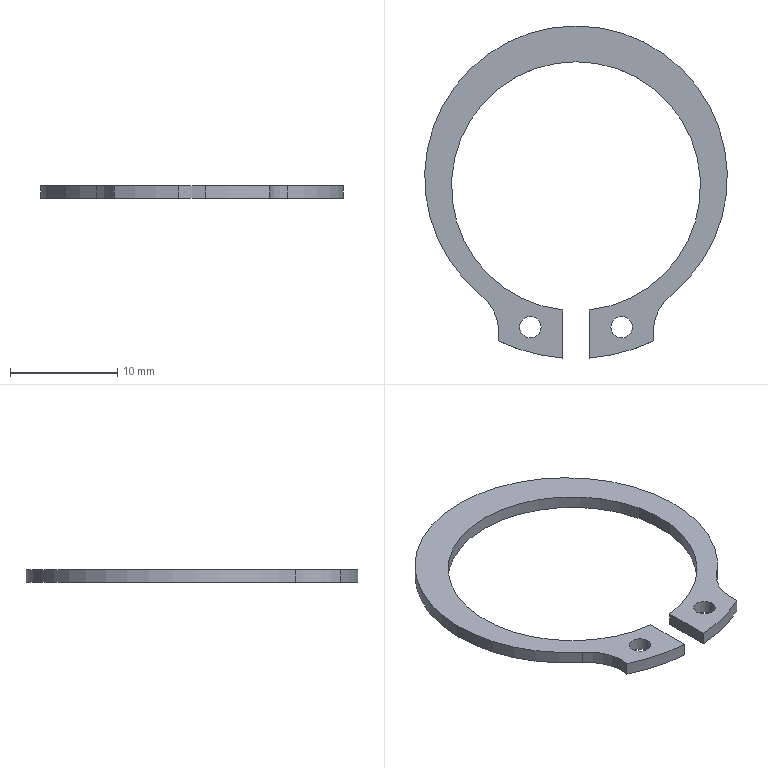Component | NX | RETAINING_RING | 1 solid | 12 faces | box 28.2 x 30.93 x 1.2 mm | volume 273 mm3 | cylinder 8 | plane 4 | commonest cylinder face diameters 2 x2 9 x2 33.76 x2 28.2 x1 23.2 x1
STEP:
#1=CARTESIAN_POINT('',(0.,0.,0.));
#2=DIRECTION('',(0.,0.,1.));
#3=DIRECTION('',(1.,0.,0.));
#4=AXIS2_PLACEMENT_3D('',#1,#2,#3);
#5=CARTESIAN_POINT('',(-594.925,295.052,-700.));
#6=VERTEX_POINT('',#5);
#7=CARTESIAN_POINT('',(-593.925,295.052,-700.));
#8=DIRECTION('',(0.,0.,1.));
#9=DIRECTION('',(-1.,0.,0.));
#10=AXIS2_PLACEMENT_3D('',#7,#8,#9);
#11=CIRCLE('',#10,1.);
#12=CARTESIAN_POINT('',(-593.925,295.052,-700.));
#13=DIRECTION('',(0.,0.,-1.));
#14=DIRECTION('',(1.,0.,0.));
#15=AXIS2_PLACEMENT_3D('',#12,#13,#14);
#16=CYLINDRICAL_SURFACE('',#15,1.);
#17=CARTESIAN_POINT('',(9.425,0.));
#18=DIRECTION('',(-1.,0.));
#19=VECTOR('',#18,1.);
#20=LINE('',#17,#19);
#21=(GEOMETRIC_REPRESENTATION_CONTEXT(2)PARAMETRIC_REPRESENTATION_CONTEXT()REPRESENTATION_CONTEXT('',''));
#22=DEFINITIONAL_REPRESENTATION('',(#20),#21);
#23=PCURVE('',#16,#22);
#24=CARTESIAN_POINT('',(-598.175,308.181,-700.));
#25=DIRECTION('',(0.,0.,1.));
#26=DIRECTION('',(-1.,0.,0.));
#27=AXIS2_PLACEMENT_3D('',#24,#25,#26);
#28=PLANE('',#27);
#29=CARTESIAN_POINT('',(-4.25,13.129));
#30=DIRECTION('',(1.,0.));
#31=AXIS2_PLACEMENT_2D('',#29,#30);
#32=CIRCLE('',#31,1.);
#33=(GEOMETRIC_REPRESENTATION_CONTEXT(2)PARAMETRIC_REPRESENTATION_CONTEXT()REPRESENTATION_CONTEXT('',''));
#34=DEFINITIONAL_REPRESENTATION('',(#32),#33);
#35=PCURVE('',#28,#34);
#36=SURFACE_CURVE('',#11,(#23,#35),.PCURVE_S1.);
#37=EDGE_CURVE('',#6,#6,#36,.T.);
#38=ORIENTED_EDGE('',*,*,#37,.F.);
#39=CARTESIAN_POINT('',(-594.925,295.052,-701.2));
#40=VERTEX_POINT('',#39);
#41=CARTESIAN_POINT('',(-594.925,295.052,-700.));
#42=CARTESIAN_POINT('',(-594.925,295.052,-701.2));
#43=B_SPLINE_CURVE_WITH_KNOTS('',1,(#41,#42),.UNSPECIFIED.,.F.,.F.,(2,2),(0.,1.2),.PIECEWISE_BEZIER_KNOTS.);
#44=CARTESIAN_POINT('',(9.425,0.));
#45=DIRECTION('',(0.,1.));
#46=VECTOR('',#45,1.);
#47=LINE('',#44,#46);
#48=(GEOMETRIC_REPRESENTATION_CONTEXT(2)PARAMETRIC_REPRESENTATION_CONTEXT()REPRESENTATION_CONTEXT('',''));
#49=DEFINITIONAL_REPRESENTATION('',(#47),#48);
#50=PCURVE('',#16,#49);
#51=CARTESIAN_POINT('',(3.142,0.));
#52=DIRECTION('',(0.,1.));
#53=VECTOR('',#52,1.);
#54=LINE('',#51,#53);
#55=(GEOMETRIC_REPRESENTATION_CONTEXT(2)PARAMETRIC_REPRESENTATION_CONTEXT()REPRESENTATION_CONTEXT('',''));
#56=DEFINITIONAL_REPRESENTATION('',(#54),#55);
#57=PCURVE('',#16,#56);
#58=SEAM_CURVE('',#43,(#50,#57),.PCURVE_S1.);
#59=EDGE_CURVE('',#6,#40,#58,.T.);
#60=ORIENTED_EDGE('',*,*,#59,.T.);
#61=CARTESIAN_POINT('',(-593.925,295.052,-701.2));
#62=DIRECTION('',(0.,0.,1.));
#63=DIRECTION('',(-1.,0.,0.));
#64=AXIS2_PLACEMENT_3D('',#61,#62,#63);
#65=CIRCLE('',#64,1.);
#66=CARTESIAN_POINT('',(9.425,1.2));
#67=DIRECTION('',(-1.,0.));
#68=VECTOR('',#67,1.);
#69=LINE('',#66,#68);
#70=(GEOMETRIC_REPRESENTATION_CONTEXT(2)PARAMETRIC_REPRESENTATION_CONTEXT()REPRESENTATION_CONTEXT('',''));
#71=DEFINITIONAL_REPRESENTATION('',(#69),#70);
#72=PCURVE('',#16,#71);
#73=CARTESIAN_POINT('',(-598.175,308.181,-701.2));
#74=DIRECTION('',(0.,0.,1.));
#75=DIRECTION('',(-1.,0.,0.));
#76=AXIS2_PLACEMENT_3D('',#73,#74,#75);
#77=PLANE('',#76);
#78=CARTESIAN_POINT('',(-4.25,13.129));
#79=DIRECTION('',(1.,0.));
#80=AXIS2_PLACEMENT_2D('',#78,#79);
#81=CIRCLE('',#80,1.);
#82=(GEOMETRIC_REPRESENTATION_CONTEXT(2)PARAMETRIC_REPRESENTATION_CONTEXT()REPRESENTATION_CONTEXT('',''));
#83=DEFINITIONAL_REPRESENTATION('',(#81),#82);
#84=PCURVE('',#77,#83);
#85=SURFACE_CURVE('',#65,(#72,#84),.PCURVE_S1.);
#86=EDGE_CURVE('',#40,#40,#85,.T.);
#87=ORIENTED_EDGE('',*,*,#86,.T.);
#88=ORIENTED_EDGE('',*,*,#59,.F.);
#89=EDGE_LOOP('',(#38,#60,#87,#88));
#90=FACE_BOUND('',#89,.F.);
#91=ADVANCED_FACE('',(#90),#16,.F.);
#92=CARTESIAN_POINT('',(-601.425,295.052,-700.));
#93=VERTEX_POINT('',#92);
#94=CARTESIAN_POINT('',(-602.425,295.052,-700.));
#95=DIRECTION('',(0.,0.,1.));
#96=DIRECTION('',(1.,0.,0.));
#97=AXIS2_PLACEMENT_3D('',#94,#95,#96);
#98=CIRCLE('',#97,1.);
#99=CARTESIAN_POINT('',(-602.425,295.052,-700.));
#100=DIRECTION('',(0.,0.,-1.));
#101=DIRECTION('',(1.,0.,0.));
#102=AXIS2_PLACEMENT_3D('',#99,#100,#101);
#103=CYLINDRICAL_SURFACE('',#102,1.);
#104=CARTESIAN_POINT('',(6.283,0.));
#105=DIRECTION('',(-1.,0.));
#106=VECTOR('',#105,1.);
#107=LINE('',#104,#106);
#108=(GEOMETRIC_REPRESENTATION_CONTEXT(2)PARAMETRIC_REPRESENTATION_CONTEXT()REPRESENTATION_CONTEXT('',''));
#109=DEFINITIONAL_REPRESENTATION('',(#107),#108);
#110=PCURVE('',#103,#109);
#111=CARTESIAN_POINT('',(4.25,13.129));
#112=DIRECTION('',(-1.,0.));
#113=AXIS2_PLACEMENT_2D('',#111,#112);
#114=CIRCLE('',#113,1.);
#115=(GEOMETRIC_REPRESENTATION_CONTEXT(2)PARAMETRIC_REPRESENTATION_CONTEXT()REPRESENTATION_CONTEXT('',''));
#116=DEFINITIONAL_REPRESENTATION('',(#114),#115);
#117=PCURVE('',#28,#116);
#118=SURFACE_CURVE('',#98,(#110,#117),.PCURVE_S1.);
#119=EDGE_CURVE('',#93,#93,#118,.T.);
#120=ORIENTED_EDGE('',*,*,#119,.F.);
#121=CARTESIAN_POINT('',(-601.425,295.052,-701.2));
#122=VERTEX_POINT('',#121);
#123=CARTESIAN_POINT('',(-601.425,295.052,-700.));
#124=CARTESIAN_POINT('',(-601.425,295.052,-701.2));
#125=B_SPLINE_CURVE_WITH_KNOTS('',1,(#123,#124),.UNSPECIFIED.,.F.,.F.,(2,2),(0.,1.2),.PIECEWISE_BEZIER_KNOTS.);
#126=CARTESIAN_POINT('',(6.283,0.));
#127=DIRECTION('',(0.,1.));
#128=VECTOR('',#127,1.);
#129=LINE('',#126,#128);
#130=(GEOMETRIC_REPRESENTATION_CONTEXT(2)PARAMETRIC_REPRESENTATION_CONTEXT()REPRESENTATION_CONTEXT('',''));
#131=DEFINITIONAL_REPRESENTATION('',(#129),#130);
#132=PCURVE('',#103,#131);
#133=CARTESIAN_POINT('',(0.,0.));
#134=DIRECTION('',(0.,1.));
#135=VECTOR('',#134,1.);
#136=LINE('',#133,#135);
#137=(GEOMETRIC_REPRESENTATION_CONTEXT(2)PARAMETRIC_REPRESENTATION_CONTEXT()REPRESENTATION_CONTEXT('',''));
#138=DEFINITIONAL_REPRESENTATION('',(#136),#137);
#139=PCURVE('',#103,#138);
#140=SEAM_CURVE('',#125,(#132,#139),.PCURVE_S1.);
#141=EDGE_CURVE('',#93,#122,#140,.T.);
#142=ORIENTED_EDGE('',*,*,#141,.T.);
#143=CARTESIAN_POINT('',(-602.425,295.052,-701.2));
#144=DIRECTION('',(0.,0.,1.));
#145=DIRECTION('',(1.,0.,0.));
#146=AXIS2_PLACEMENT_3D('',#143,#144,#145);
#147=CIRCLE('',#146,1.);
#148=CARTESIAN_POINT('',(6.283,1.2));
#149=DIRECTION('',(-1.,0.));
#150=VECTOR('',#149,1.);
#151=LINE('',#148,#150);
#152=(GEOMETRIC_REPRESENTATION_CONTEXT(2)PARAMETRIC_REPRESENTATION_CONTEXT()REPRESENTATION_CONTEXT('',''));
#153=DEFINITIONAL_REPRESENTATION('',(#151),#152);
#154=PCURVE('',#103,#153);
#155=CARTESIAN_POINT('',(4.25,13.129));
#156=DIRECTION('',(-1.,0.));
#157=AXIS2_PLACEMENT_2D('',#155,#156);
#158=CIRCLE('',#157,1.);
#159=(GEOMETRIC_REPRESENTATION_CONTEXT(2)PARAMETRIC_REPRESENTATION_CONTEXT()REPRESENTATION_CONTEXT('',''));
#160=DEFINITIONAL_REPRESENTATION('',(#158),#159);
#161=PCURVE('',#77,#160);
#162=SURFACE_CURVE('',#147,(#154,#161),.PCURVE_S1.);
#163=EDGE_CURVE('',#122,#122,#162,.T.);
#164=ORIENTED_EDGE('',*,*,#163,.T.);
#165=ORIENTED_EDGE('',*,*,#141,.F.);
#166=EDGE_LOOP('',(#120,#142,#164,#165));
#167=FACE_BOUND('',#166,.F.);
#168=ADVANCED_FACE('',(#167),#103,.F.);
#169=CARTESIAN_POINT('',(-589.318,298.04,-700.));
#170=VERTEX_POINT('',#169);
#171=CARTESIAN_POINT('',(-607.032,298.04,-700.));
#172=VERTEX_POINT('',#171);
#173=CARTESIAN_POINT('',(-598.175,309.011,-700.));
#174=DIRECTION('',(0.,0.,1.));
#175=DIRECTION('',(1.,0.,0.));
#176=AXIS2_PLACEMENT_3D('',#173,#174,#175);
#177=CIRCLE('',#176,14.1);
#178=CARTESIAN_POINT('',(-598.175,309.011,-700.));
#179=DIRECTION('',(0.,0.,-1.));
#180=DIRECTION('',(1.,0.,0.));
#181=AXIS2_PLACEMENT_3D('',#178,#179,#180);
#182=CYLINDRICAL_SURFACE('',#181,14.1);
#183=CARTESIAN_POINT('',(12.566,0.));
#184=DIRECTION('',(-1.,0.));
#185=VECTOR('',#184,1.);
#186=LINE('',#183,#185);
#187=(GEOMETRIC_REPRESENTATION_CONTEXT(2)PARAMETRIC_REPRESENTATION_CONTEXT()REPRESENTATION_CONTEXT('',''));
#188=DEFINITIONAL_REPRESENTATION('',(#186),#187);
#189=PCURVE('',#182,#188);
#190=CARTESIAN_POINT('',(0.,-0.83));
#191=DIRECTION('',(-1.,0.));
#192=AXIS2_PLACEMENT_2D('',#190,#191);
#193=CIRCLE('',#192,14.1);
#194=(GEOMETRIC_REPRESENTATION_CONTEXT(2)PARAMETRIC_REPRESENTATION_CONTEXT()REPRESENTATION_CONTEXT('',''));
#195=DEFINITIONAL_REPRESENTATION('',(#193),#194);
#196=PCURVE('',#28,#195);
#197=SURFACE_CURVE('',#177,(#189,#196),.PCURVE_S1.);
#198=EDGE_CURVE('',#170,#172,#197,.T.);
#199=ORIENTED_EDGE('',*,*,#198,.F.);
#200=CARTESIAN_POINT('',(-589.318,298.04,-701.2));
#201=VERTEX_POINT('',#200);
#202=CARTESIAN_POINT('',(-589.318,298.04,-700.));
#203=DIRECTION('',(0.,0.,-1.));
#204=VECTOR('',#203,1.);
#205=LINE('',#202,#204);
#206=CARTESIAN_POINT('',(7.175,0.));
#207=DIRECTION('',(0.,1.));
#208=VECTOR('',#207,1.);
#209=LINE('',#206,#208);
#210=(GEOMETRIC_REPRESENTATION_CONTEXT(2)PARAMETRIC_REPRESENTATION_CONTEXT()REPRESENTATION_CONTEXT('',''));
#211=DEFINITIONAL_REPRESENTATION('',(#209),#210);
#212=PCURVE('',#182,#211);
#213=CARTESIAN_POINT('',(-586.492,294.539,-700.));
#214=DIRECTION('',(0.,0.,-1.));
#215=DIRECTION('',(1.,0.,0.));
#216=AXIS2_PLACEMENT_3D('',#213,#214,#215);
#217=CYLINDRICAL_SURFACE('',#216,4.5);
#218=CARTESIAN_POINT('',(4.033,0.));
#219=DIRECTION('',(0.,1.));
#220=VECTOR('',#219,1.);
#221=LINE('',#218,#220);
#222=(GEOMETRIC_REPRESENTATION_CONTEXT(2)PARAMETRIC_REPRESENTATION_CONTEXT()REPRESENTATION_CONTEXT('',''));
#223=DEFINITIONAL_REPRESENTATION('',(#221),#222);
#224=PCURVE('',#217,#223);
#225=SURFACE_CURVE('',#205,(#212,#224),.PCURVE_S1.);
#226=EDGE_CURVE('',#170,#201,#225,.T.);
#227=ORIENTED_EDGE('',*,*,#226,.T.);
#228=CARTESIAN_POINT('',(-607.032,298.04,-701.2));
#229=VERTEX_POINT('',#228);
#230=CARTESIAN_POINT('',(-598.175,309.011,-701.2));
#231=DIRECTION('',(0.,0.,1.));
#232=DIRECTION('',(1.,0.,0.));
#233=AXIS2_PLACEMENT_3D('',#230,#231,#232);
#234=CIRCLE('',#233,14.1);
#235=CARTESIAN_POINT('',(12.566,1.2));
#236=DIRECTION('',(-1.,0.));
#237=VECTOR('',#236,1.);
#238=LINE('',#235,#237);
#239=(GEOMETRIC_REPRESENTATION_CONTEXT(2)PARAMETRIC_REPRESENTATION_CONTEXT()REPRESENTATION_CONTEXT('',''));
#240=DEFINITIONAL_REPRESENTATION('',(#238),#239);
#241=PCURVE('',#182,#240);
#242=CARTESIAN_POINT('',(0.,-0.83));
#243=DIRECTION('',(-1.,0.));
#244=AXIS2_PLACEMENT_2D('',#242,#243);
#245=CIRCLE('',#244,14.1);
#246=(GEOMETRIC_REPRESENTATION_CONTEXT(2)PARAMETRIC_REPRESENTATION_CONTEXT()REPRESENTATION_CONTEXT('',''));
#247=DEFINITIONAL_REPRESENTATION('',(#245),#246);
#248=PCURVE('',#77,#247);
#249=SURFACE_CURVE('',#234,(#241,#248),.PCURVE_S1.);
#250=EDGE_CURVE('',#201,#229,#249,.T.);
#251=ORIENTED_EDGE('',*,*,#250,.T.);
#252=CARTESIAN_POINT('',(-607.032,298.04,-700.));
#253=DIRECTION('',(0.,0.,-1.));
#254=VECTOR('',#253,1.);
#255=LINE('',#252,#254);
#256=CARTESIAN_POINT('',(2.25,0.));
#257=DIRECTION('',(0.,1.));
#258=VECTOR('',#257,1.);
#259=LINE('',#256,#258);
#260=(GEOMETRIC_REPRESENTATION_CONTEXT(2)PARAMETRIC_REPRESENTATION_CONTEXT()REPRESENTATION_CONTEXT('',''));
#261=DEFINITIONAL_REPRESENTATION('',(#259),#260);
#262=PCURVE('',#182,#261);
#263=CARTESIAN_POINT('',(-609.859,294.539,-700.));
#264=DIRECTION('',(0.,0.,-1.));
#265=DIRECTION('',(1.,0.,0.));
#266=AXIS2_PLACEMENT_3D('',#263,#264,#265);
#267=CYLINDRICAL_SURFACE('',#266,4.5);
#268=CARTESIAN_POINT('',(5.392,0.));
#269=DIRECTION('',(0.,1.));
#270=VECTOR('',#269,1.);
#271=LINE('',#268,#270);
#272=(GEOMETRIC_REPRESENTATION_CONTEXT(2)PARAMETRIC_REPRESENTATION_CONTEXT()REPRESENTATION_CONTEXT('',''));
#273=DEFINITIONAL_REPRESENTATION('',(#271),#272);
#274=PCURVE('',#267,#273);
#275=SURFACE_CURVE('',#255,(#262,#274),.PCURVE_S1.);
#276=EDGE_CURVE('',#172,#229,#275,.T.);
#277=ORIENTED_EDGE('',*,*,#276,.F.);
#278=EDGE_LOOP('',(#199,#227,#251,#277));
#279=FACE_BOUND('',#278,.T.);
#280=ADVANCED_FACE('',(#279),#182,.T.);
#281=ORIENTED_EDGE('',*,*,#226,.T.);
#282=CARTESIAN_POINT('',(-590.925,293.768,-701.2));
#283=VERTEX_POINT('',#282);
#284=CARTESIAN_POINT('',(-586.492,294.539,-701.2));
#285=DIRECTION('',(0.,0.,-1.));
#286=DIRECTION('',(-1.,0.,0.));
#287=AXIS2_PLACEMENT_3D('',#284,#285,#286);
#288=CIRCLE('',#287,4.5);
#289=CARTESIAN_POINT('',(-3.142,1.2));
#290=DIRECTION('',(1.,0.));
#291=VECTOR('',#290,1.);
#292=LINE('',#289,#291);
#293=(GEOMETRIC_REPRESENTATION_CONTEXT(2)PARAMETRIC_REPRESENTATION_CONTEXT()REPRESENTATION_CONTEXT('',''));
#294=DEFINITIONAL_REPRESENTATION('',(#292),#293);
#295=PCURVE('',#217,#294);
#296=CARTESIAN_POINT('',(-7.183,13.643));
#297=CARTESIAN_POINT('',(-7.183,5.848));
#298=CARTESIAN_POINT('',(-13.933,9.746));
#299=CARTESIAN_POINT('',(-20.683,13.643));
#300=CARTESIAN_POINT('',(-13.933,17.54));
#301=CARTESIAN_POINT('',(-7.183,21.437));
#302=CARTESIAN_POINT('',(-7.183,13.643));
#303=(BOUNDED_CURVE()B_SPLINE_CURVE(2,(#296,#297,#298,#299,#300,#301,#302),.UNSPECIFIED.,.T.,.F.)B_SPLINE_CURVE_WITH_KNOTS((1,2,2,2,2,1),(-2.094,0.,2.094,4.189,6.283,8.378),.UNSPECIFIED.)CURVE()GEOMETRIC_REPRESENTATION_ITEM()RATIONAL_B_SPLINE_CURVE((1.,0.5,1.,0.5,1.,0.5,1.))REPRESENTATION_ITEM(''));
#304=(GEOMETRIC_REPRESENTATION_CONTEXT(2)PARAMETRIC_REPRESENTATION_CONTEXT()REPRESENTATION_CONTEXT('',''));
#305=DEFINITIONAL_REPRESENTATION('',(#303),#304);
#306=PCURVE('',#77,#305);
#307=SURFACE_CURVE('',#288,(#295,#306),.PCURVE_S1.);
#308=EDGE_CURVE('',#283,#201,#307,.T.);
#309=ORIENTED_EDGE('',*,*,#308,.F.);
#310=CARTESIAN_POINT('',(-590.925,293.768,-700.));
#311=VERTEX_POINT('',#310);
#312=CARTESIAN_POINT('',(-590.925,293.768,-700.));
#313=DIRECTION('',(0.,0.,-1.));
#314=VECTOR('',#313,1.);
#315=LINE('',#312,#314);
#316=CARTESIAN_POINT('',(2.969,0.));
#317=DIRECTION('',(0.,1.));
#318=VECTOR('',#317,1.);
#319=LINE('',#316,#318);
#320=(GEOMETRIC_REPRESENTATION_CONTEXT(2)PARAMETRIC_REPRESENTATION_CONTEXT()REPRESENTATION_CONTEXT('',''));
#321=DEFINITIONAL_REPRESENTATION('',(#319),#320);
#322=PCURVE('',#217,#321);
#323=CARTESIAN_POINT('',(-598.175,309.011,-700.));
#324=DIRECTION('',(0.,0.,-1.));
#325=DIRECTION('',(1.,0.,0.));
#326=AXIS2_PLACEMENT_3D('',#323,#324,#325);
#327=CYLINDRICAL_SURFACE('',#326,16.88);
#328=CARTESIAN_POINT('',(1.127,0.));
#329=DIRECTION('',(0.,1.));
#330=VECTOR('',#329,1.);
#331=LINE('',#328,#330);
#332=(GEOMETRIC_REPRESENTATION_CONTEXT(2)PARAMETRIC_REPRESENTATION_CONTEXT()REPRESENTATION_CONTEXT('',''));
#333=DEFINITIONAL_REPRESENTATION('',(#331),#332);
#334=PCURVE('',#327,#333);
#335=SURFACE_CURVE('',#315,(#322,#334),.PCURVE_S1.);
#336=EDGE_CURVE('',#311,#283,#335,.T.);
#337=ORIENTED_EDGE('',*,*,#336,.F.);
#338=CARTESIAN_POINT('',(-586.492,294.539,-700.));
#339=DIRECTION('',(0.,0.,-1.));
#340=DIRECTION('',(-1.,0.,0.));
#341=AXIS2_PLACEMENT_3D('',#338,#339,#340);
#342=CIRCLE('',#341,4.5);
#343=CARTESIAN_POINT('',(-3.142,0.));
#344=DIRECTION('',(1.,0.));
#345=VECTOR('',#344,1.);
#346=LINE('',#343,#345);
#347=(GEOMETRIC_REPRESENTATION_CONTEXT(2)PARAMETRIC_REPRESENTATION_CONTEXT()REPRESENTATION_CONTEXT('',''));
#348=DEFINITIONAL_REPRESENTATION('',(#346),#347);
#349=PCURVE('',#217,#348);
#350=CARTESIAN_POINT('',(-7.183,13.643));
#351=CARTESIAN_POINT('',(-7.183,5.848));
#352=CARTESIAN_POINT('',(-13.933,9.746));
#353=CARTESIAN_POINT('',(-20.683,13.643));
#354=CARTESIAN_POINT('',(-13.933,17.54));
#355=CARTESIAN_POINT('',(-7.183,21.437));
#356=CARTESIAN_POINT('',(-7.183,13.643));
#357=(BOUNDED_CURVE()B_SPLINE_CURVE(2,(#350,#351,#352,#353,#354,#355,#356),.UNSPECIFIED.,.T.,.F.)B_SPLINE_CURVE_WITH_KNOTS((1,2,2,2,2,1),(-2.094,0.,2.094,4.189,6.283,8.378),.UNSPECIFIED.)CURVE()GEOMETRIC_REPRESENTATION_ITEM()RATIONAL_B_SPLINE_CURVE((1.,0.5,1.,0.5,1.,0.5,1.))REPRESENTATION_ITEM(''));
#358=(GEOMETRIC_REPRESENTATION_CONTEXT(2)PARAMETRIC_REPRESENTATION_CONTEXT()REPRESENTATION_CONTEXT('',''));
#359=DEFINITIONAL_REPRESENTATION('',(#357),#358);
#360=PCURVE('',#28,#359);
#361=SURFACE_CURVE('',#342,(#349,#360),.PCURVE_S1.);
#362=EDGE_CURVE('',#311,#170,#361,.T.);
#363=ORIENTED_EDGE('',*,*,#362,.T.);
#364=EDGE_LOOP('',(#281,#309,#337,#363));
#365=FACE_BOUND('',#364,.F.);
#366=ADVANCED_FACE('',(#365),#217,.F.);
#367=CARTESIAN_POINT('',(-596.925,296.649,-700.));
#368=VERTEX_POINT('',#367);
#369=CARTESIAN_POINT('',(-596.925,296.649,-701.2));
#370=VERTEX_POINT('',#369);
#371=CARTESIAN_POINT('',(-596.925,296.649,-700.));
#372=DIRECTION('',(0.,0.,-1.));
#373=VECTOR('',#372,1.);
#374=LINE('',#371,#373);
#375=CARTESIAN_POINT('',(-598.175,308.181,-700.));
#376=DIRECTION('',(0.,0.,-1.));
#377=DIRECTION('',(1.,0.,0.));
#378=AXIS2_PLACEMENT_3D('',#375,#376,#377);
#379=CYLINDRICAL_SURFACE('',#378,11.6);
#380=CARTESIAN_POINT('',(7.746,0.));
#381=DIRECTION('',(0.,1.));
#382=VECTOR('',#381,1.);
#383=LINE('',#380,#382);
#384=(GEOMETRIC_REPRESENTATION_CONTEXT(2)PARAMETRIC_REPRESENTATION_CONTEXT()REPRESENTATION_CONTEXT('',''));
#385=DEFINITIONAL_REPRESENTATION('',(#383),#384);
#386=PCURVE('',#379,#385);
#387=CARTESIAN_POINT('',(-596.925,296.649,-700.));
#388=DIRECTION('',(1.,0.,0.));
#389=DIRECTION('',(0.,-1.,0.));
#390=AXIS2_PLACEMENT_3D('',#387,#388,#389);
#391=PLANE('',#390);
#392=CARTESIAN_POINT('',(0.,0.));
#393=DIRECTION('',(0.,1.));
#394=VECTOR('',#393,1.);
#395=LINE('',#392,#394);
#396=(GEOMETRIC_REPRESENTATION_CONTEXT(2)PARAMETRIC_REPRESENTATION_CONTEXT()REPRESENTATION_CONTEXT('',''));
#397=DEFINITIONAL_REPRESENTATION('',(#395),#396);
#398=PCURVE('',#391,#397);
#399=SURFACE_CURVE('',#374,(#386,#398),.PCURVE_S1.);
#400=EDGE_CURVE('',#368,#370,#399,.T.);
#401=ORIENTED_EDGE('',*,*,#400,.T.);
#402=CARTESIAN_POINT('',(-599.425,296.649,-701.2));
#403=VERTEX_POINT('',#402);
#404=CARTESIAN_POINT('',(-598.175,308.181,-701.2));
#405=DIRECTION('',(0.,0.,-1.));
#406=DIRECTION('',(1.,0.,0.));
#407=AXIS2_PLACEMENT_3D('',#404,#405,#406);
#408=CIRCLE('',#407,11.6);
#409=CARTESIAN_POINT('',(-0.,1.2));
#410=DIRECTION('',(1.,0.));
#411=VECTOR('',#410,1.);
#412=LINE('',#409,#411);
#413=(GEOMETRIC_REPRESENTATION_CONTEXT(2)PARAMETRIC_REPRESENTATION_CONTEXT()REPRESENTATION_CONTEXT('',''));
#414=DEFINITIONAL_REPRESENTATION('',(#412),#413);
#415=PCURVE('',#379,#414);
#416=CARTESIAN_POINT('',(-11.6,0.));
#417=CARTESIAN_POINT('',(-11.6,20.092));
#418=CARTESIAN_POINT('',(5.8,10.046));
#419=CARTESIAN_POINT('',(23.2,0.));
#420=CARTESIAN_POINT('',(5.8,-10.046));
#421=CARTESIAN_POINT('',(-11.6,-20.092));
#422=CARTESIAN_POINT('',(-11.6,0.));
#423=(BOUNDED_CURVE()B_SPLINE_CURVE(2,(#416,#417,#418,#419,#420,#421,#422),.UNSPECIFIED.,.T.,.F.)B_SPLINE_CURVE_WITH_KNOTS((1,2,2,2,2,1),(-2.094,0.,2.094,4.189,6.283,8.378),.UNSPECIFIED.)CURVE()GEOMETRIC_REPRESENTATION_ITEM()RATIONAL_B_SPLINE_CURVE((1.,0.5,1.,0.5,1.,0.5,1.))REPRESENTATION_ITEM(''));
#424=(GEOMETRIC_REPRESENTATION_CONTEXT(2)PARAMETRIC_REPRESENTATION_CONTEXT()REPRESENTATION_CONTEXT('',''));
#425=DEFINITIONAL_REPRESENTATION('',(#423),#424);
#426=PCURVE('',#77,#425);
#427=SURFACE_CURVE('',#408,(#415,#426),.PCURVE_S1.);
#428=EDGE_CURVE('',#403,#370,#427,.T.);
#429=ORIENTED_EDGE('',*,*,#428,.F.);
#430=CARTESIAN_POINT('',(-599.425,296.649,-700.));
#431=VERTEX_POINT('',#430);
#432=CARTESIAN_POINT('',(-599.425,296.649,-700.));
#433=DIRECTION('',(0.,0.,-1.));
#434=VECTOR('',#433,1.);
#435=LINE('',#432,#434);
#436=CARTESIAN_POINT('',(1.679,0.));
#437=DIRECTION('',(0.,1.));
#438=VECTOR('',#437,1.);
#439=LINE('',#436,#438);
#440=(GEOMETRIC_REPRESENTATION_CONTEXT(2)PARAMETRIC_REPRESENTATION_CONTEXT()REPRESENTATION_CONTEXT('',''));
#441=DEFINITIONAL_REPRESENTATION('',(#439),#440);
#442=PCURVE('',#379,#441);
#443=CARTESIAN_POINT('',(-599.425,296.649,-700.));
#444=DIRECTION('',(-1.,-0.,0.));
#445=DIRECTION('',(-0.,1.,0.));
#446=AXIS2_PLACEMENT_3D('',#443,#444,#445);
#447=PLANE('',#446);
#448=CARTESIAN_POINT('',(0.,0.));
#449=DIRECTION('',(0.,1.));
#450=VECTOR('',#449,1.);
#451=LINE('',#448,#450);
#452=(GEOMETRIC_REPRESENTATION_CONTEXT(2)PARAMETRIC_REPRESENTATION_CONTEXT()REPRESENTATION_CONTEXT('',''));
#453=DEFINITIONAL_REPRESENTATION('',(#451),#452);
#454=PCURVE('',#447,#453);
#455=SURFACE_CURVE('',#435,(#442,#454),.PCURVE_S1.);
#456=EDGE_CURVE('',#431,#403,#455,.T.);
#457=ORIENTED_EDGE('',*,*,#456,.F.);
#458=CARTESIAN_POINT('',(-598.175,308.181,-700.));
#459=DIRECTION('',(0.,0.,-1.));
#460=DIRECTION('',(1.,0.,0.));
#461=AXIS2_PLACEMENT_3D('',#458,#459,#460);
#462=CIRCLE('',#461,11.6);
#463=CARTESIAN_POINT('',(-0.,0.));
#464=DIRECTION('',(1.,0.));
#465=VECTOR('',#464,1.);
#466=LINE('',#463,#465);
#467=(GEOMETRIC_REPRESENTATION_CONTEXT(2)PARAMETRIC_REPRESENTATION_CONTEXT()REPRESENTATION_CONTEXT('',''));
#468=DEFINITIONAL_REPRESENTATION('',(#466),#467);
#469=PCURVE('',#379,#468);
#470=CARTESIAN_POINT('',(-11.6,0.));
#471=CARTESIAN_POINT('',(-11.6,20.092));
#472=CARTESIAN_POINT('',(5.8,10.046));
#473=CARTESIAN_POINT('',(23.2,0.));
#474=CARTESIAN_POINT('',(5.8,-10.046));
#475=CARTESIAN_POINT('',(-11.6,-20.092));
#476=CARTESIAN_POINT('',(-11.6,0.));
#477=(BOUNDED_CURVE()B_SPLINE_CURVE(2,(#470,#471,#472,#473,#474,#475,#476),.UNSPECIFIED.,.T.,.F.)B_SPLINE_CURVE_WITH_KNOTS((1,2,2,2,2,1),(-2.094,0.,2.094,4.189,6.283,8.378),.UNSPECIFIED.)CURVE()GEOMETRIC_REPRESENTATION_ITEM()RATIONAL_B_SPLINE_CURVE((1.,0.5,1.,0.5,1.,0.5,1.))REPRESENTATION_ITEM(''));
#478=(GEOMETRIC_REPRESENTATION_CONTEXT(2)PARAMETRIC_REPRESENTATION_CONTEXT()REPRESENTATION_CONTEXT('',''));
#479=DEFINITIONAL_REPRESENTATION('',(#477),#478);
#480=PCURVE('',#28,#479);
#481=SURFACE_CURVE('',#462,(#469,#480),.PCURVE_S1.);
#482=EDGE_CURVE('',#431,#368,#481,.T.);
#483=ORIENTED_EDGE('',*,*,#482,.T.);
#484=EDGE_LOOP('',(#401,#429,#457,#483));
#485=FACE_BOUND('',#484,.F.);
#486=ADVANCED_FACE('',(#485),#379,.F.);
#487=ORIENTED_EDGE('',*,*,#119,.F.);
#488=EDGE_LOOP('',(#487));
#489=FACE_BOUND('',#488,.T.);
#490=CARTESIAN_POINT('',(-599.425,292.178,-700.));
#491=VERTEX_POINT('',#490);
#492=CARTESIAN_POINT('',(-599.425,296.649,-700.));
#493=DIRECTION('',(-0.,1.,0.));
#494=VECTOR('',#493,1.);
#495=LINE('',#492,#494);
#496=CARTESIAN_POINT('',(1.25,11.532));
#497=DIRECTION('',(0.,-1.));
#498=VECTOR('',#497,1.);
#499=LINE('',#496,#498);
#500=(GEOMETRIC_REPRESENTATION_CONTEXT(2)PARAMETRIC_REPRESENTATION_CONTEXT()REPRESENTATION_CONTEXT('',''));
#501=DEFINITIONAL_REPRESENTATION('',(#499),#500);
#502=PCURVE('',#28,#501);
#503=CARTESIAN_POINT('',(0.,0.));
#504=DIRECTION('',(1.,0.));
#505=VECTOR('',#504,1.);
#506=LINE('',#503,#505);
#507=(GEOMETRIC_REPRESENTATION_CONTEXT(2)PARAMETRIC_REPRESENTATION_CONTEXT()REPRESENTATION_CONTEXT('',''));
#508=DEFINITIONAL_REPRESENTATION('',(#506),#507);
#509=PCURVE('',#447,#508);
#510=SURFACE_CURVE('',#495,(#502,#509),.PCURVE_S1.);
#511=EDGE_CURVE('',#491,#431,#510,.T.);
#512=ORIENTED_EDGE('',*,*,#511,.T.);
#513=ORIENTED_EDGE('',*,*,#482,.T.);
#514=CARTESIAN_POINT('',(-596.925,292.178,-700.));
#515=VERTEX_POINT('',#514);
#516=CARTESIAN_POINT('',(-596.925,296.649,-700.));
#517=DIRECTION('',(0.,-1.,0.));
#518=VECTOR('',#517,1.);
#519=LINE('',#516,#518);
#520=CARTESIAN_POINT('',(-1.25,11.532));
#521=DIRECTION('',(-0.,1.));
#522=VECTOR('',#521,1.);
#523=LINE('',#520,#522);
#524=(GEOMETRIC_REPRESENTATION_CONTEXT(2)PARAMETRIC_REPRESENTATION_CONTEXT()REPRESENTATION_CONTEXT('',''));
#525=DEFINITIONAL_REPRESENTATION('',(#523),#524);
#526=PCURVE('',#28,#525);
#527=CARTESIAN_POINT('',(0.,0.));
#528=DIRECTION('',(1.,0.));
#529=VECTOR('',#528,1.);
#530=LINE('',#527,#529);
#531=(GEOMETRIC_REPRESENTATION_CONTEXT(2)PARAMETRIC_REPRESENTATION_CONTEXT()REPRESENTATION_CONTEXT('',''));
#532=DEFINITIONAL_REPRESENTATION('',(#530),#531);
#533=PCURVE('',#391,#532);
#534=SURFACE_CURVE('',#519,(#526,#533),.PCURVE_S1.);
#535=EDGE_CURVE('',#368,#515,#534,.T.);
#536=ORIENTED_EDGE('',*,*,#535,.T.);
#537=CARTESIAN_POINT('',(-598.175,309.011,-700.));
#538=DIRECTION('',(0.,0.,1.));
#539=DIRECTION('',(1.,0.,0.));
#540=AXIS2_PLACEMENT_3D('',#537,#538,#539);
#541=CIRCLE('',#540,16.88);
#542=CARTESIAN_POINT('',(0.,-0.83));
#543=DIRECTION('',(-1.,0.));
#544=AXIS2_PLACEMENT_2D('',#542,#543);
#545=CIRCLE('',#544,16.88);
#546=(GEOMETRIC_REPRESENTATION_CONTEXT(2)PARAMETRIC_REPRESENTATION_CONTEXT()REPRESENTATION_CONTEXT('',''));
#547=DEFINITIONAL_REPRESENTATION('',(#545),#546);
#548=PCURVE('',#28,#547);
#549=CARTESIAN_POINT('',(6.283,0.));
#550=DIRECTION('',(-1.,0.));
#551=VECTOR('',#550,1.);
#552=LINE('',#549,#551);
#553=(GEOMETRIC_REPRESENTATION_CONTEXT(2)PARAMETRIC_REPRESENTATION_CONTEXT()REPRESENTATION_CONTEXT('',''));
#554=DEFINITIONAL_REPRESENTATION('',(#552),#553);
#555=PCURVE('',#327,#554);
#556=SURFACE_CURVE('',#541,(#548,#555),.PCURVE_S1.);
#557=EDGE_CURVE('',#515,#311,#556,.T.);
#558=ORIENTED_EDGE('',*,*,#557,.T.);
#559=ORIENTED_EDGE('',*,*,#362,.T.);
#560=ORIENTED_EDGE('',*,*,#198,.T.);
#561=CARTESIAN_POINT('',(-605.425,293.768,-700.));
#562=VERTEX_POINT('',#561);
#563=CARTESIAN_POINT('',(-609.859,294.539,-700.));
#564=DIRECTION('',(0.,0.,-1.));
#565=DIRECTION('',(1.,0.,0.));
#566=AXIS2_PLACEMENT_3D('',#563,#564,#565);
#567=CIRCLE('',#566,4.5);
#568=CARTESIAN_POINT('',(7.183,13.643));
#569=CARTESIAN_POINT('',(7.183,21.437));
#570=CARTESIAN_POINT('',(13.933,17.54));
#571=CARTESIAN_POINT('',(20.683,13.643));
#572=CARTESIAN_POINT('',(13.933,9.746));
#573=CARTESIAN_POINT('',(7.183,5.848));
#574=CARTESIAN_POINT('',(7.183,13.643));
#575=(BOUNDED_CURVE()B_SPLINE_CURVE(2,(#568,#569,#570,#571,#572,#573,#574),.UNSPECIFIED.,.T.,.F.)B_SPLINE_CURVE_WITH_KNOTS((1,2,2,2,2,1),(-2.094,0.,2.094,4.189,6.283,8.378),.UNSPECIFIED.)CURVE()GEOMETRIC_REPRESENTATION_ITEM()RATIONAL_B_SPLINE_CURVE((1.,0.5,1.,0.5,1.,0.5,1.))REPRESENTATION_ITEM(''));
#576=(GEOMETRIC_REPRESENTATION_CONTEXT(2)PARAMETRIC_REPRESENTATION_CONTEXT()REPRESENTATION_CONTEXT('',''));
#577=DEFINITIONAL_REPRESENTATION('',(#575),#576);
#578=PCURVE('',#28,#577);
#579=CARTESIAN_POINT('',(0.,0.));
#580=DIRECTION('',(1.,0.));
#581=VECTOR('',#580,1.);
#582=LINE('',#579,#581);
#583=(GEOMETRIC_REPRESENTATION_CONTEXT(2)PARAMETRIC_REPRESENTATION_CONTEXT()REPRESENTATION_CONTEXT('',''));
#584=DEFINITIONAL_REPRESENTATION('',(#582),#583);
#585=PCURVE('',#267,#584);
#586=SURFACE_CURVE('',#567,(#578,#585),.PCURVE_S1.);
#587=EDGE_CURVE('',#172,#562,#586,.T.);
#588=ORIENTED_EDGE('',*,*,#587,.T.);
#589=CARTESIAN_POINT('',(-598.175,309.011,-700.));
#590=DIRECTION('',(0.,0.,1.));
#591=DIRECTION('',(-1.,0.,0.));
#592=AXIS2_PLACEMENT_3D('',#589,#590,#591);
#593=CIRCLE('',#592,16.88);
#594=CARTESIAN_POINT('',(0.,-0.83));
#595=DIRECTION('',(1.,0.));
#596=AXIS2_PLACEMENT_2D('',#594,#595);
#597=CIRCLE('',#596,16.88);
#598=(GEOMETRIC_REPRESENTATION_CONTEXT(2)PARAMETRIC_REPRESENTATION_CONTEXT()REPRESENTATION_CONTEXT('',''));
#599=DEFINITIONAL_REPRESENTATION('',(#597),#598);
#600=PCURVE('',#28,#599);
#601=CARTESIAN_POINT('',(-598.175,309.011,-700.));
#602=DIRECTION('',(0.,0.,-1.));
#603=DIRECTION('',(1.,0.,0.));
#604=AXIS2_PLACEMENT_3D('',#601,#602,#603);
#605=CYLINDRICAL_SURFACE('',#604,16.88);
#606=CARTESIAN_POINT('',(3.142,0.));
#607=DIRECTION('',(-1.,0.));
#608=VECTOR('',#607,1.);
#609=LINE('',#606,#608);
#610=(GEOMETRIC_REPRESENTATION_CONTEXT(2)PARAMETRIC_REPRESENTATION_CONTEXT()REPRESENTATION_CONTEXT('',''));
#611=DEFINITIONAL_REPRESENTATION('',(#609),#610);
#612=PCURVE('',#605,#611);
#613=SURFACE_CURVE('',#593,(#600,#612),.PCURVE_S1.);
#614=EDGE_CURVE('',#562,#491,#613,.T.);
#615=ORIENTED_EDGE('',*,*,#614,.T.);
#616=EDGE_LOOP('',(#512,#513,#536,#558,#559,#560,#588,#615));
#617=FACE_BOUND('',#616,.T.);
#618=ORIENTED_EDGE('',*,*,#37,.F.);
#619=EDGE_LOOP('',(#618));
#620=FACE_BOUND('',#619,.T.);
#621=ADVANCED_FACE('',(#489,#617,#620),#28,.T.);
#622=ORIENTED_EDGE('',*,*,#400,.T.);
#623=CARTESIAN_POINT('',(-596.925,292.178,-701.2));
#624=VERTEX_POINT('',#623);
#625=CARTESIAN_POINT('',(-596.925,296.649,-701.2));
#626=DIRECTION('',(0.,-1.,0.));
#627=VECTOR('',#626,1.);
#628=LINE('',#625,#627);
#629=CARTESIAN_POINT('',(0.,1.2));
#630=DIRECTION('',(1.,0.));
#631=VECTOR('',#630,1.);
#632=LINE('',#629,#631);
#633=(GEOMETRIC_REPRESENTATION_CONTEXT(2)PARAMETRIC_REPRESENTATION_CONTEXT()REPRESENTATION_CONTEXT('',''));
#634=DEFINITIONAL_REPRESENTATION('',(#632),#633);
#635=PCURVE('',#391,#634);
#636=CARTESIAN_POINT('',(-1.25,11.532));
#637=DIRECTION('',(-0.,1.));
#638=VECTOR('',#637,1.);
#639=LINE('',#636,#638);
#640=(GEOMETRIC_REPRESENTATION_CONTEXT(2)PARAMETRIC_REPRESENTATION_CONTEXT()REPRESENTATION_CONTEXT('',''));
#641=DEFINITIONAL_REPRESENTATION('',(#639),#640);
#642=PCURVE('',#77,#641);
#643=SURFACE_CURVE('',#628,(#635,#642),.PCURVE_S1.);
#644=EDGE_CURVE('',#370,#624,#643,.T.);
#645=ORIENTED_EDGE('',*,*,#644,.T.);
#646=CARTESIAN_POINT('',(-596.925,292.178,-700.));
#647=DIRECTION('',(0.,0.,-1.));
#648=VECTOR('',#647,1.);
#649=LINE('',#646,#648);
#650=CARTESIAN_POINT('',(4.471,0.));
#651=DIRECTION('',(0.,1.));
#652=VECTOR('',#651,1.);
#653=LINE('',#650,#652);
#654=(GEOMETRIC_REPRESENTATION_CONTEXT(2)PARAMETRIC_REPRESENTATION_CONTEXT()REPRESENTATION_CONTEXT('',''));
#655=DEFINITIONAL_REPRESENTATION('',(#653),#654);
#656=PCURVE('',#391,#655);
#657=CARTESIAN_POINT('',(1.497,0.));
#658=DIRECTION('',(0.,1.));
#659=VECTOR('',#658,1.);
#660=LINE('',#657,#659);
#661=(GEOMETRIC_REPRESENTATION_CONTEXT(2)PARAMETRIC_REPRESENTATION_CONTEXT()REPRESENTATION_CONTEXT('',''));
#662=DEFINITIONAL_REPRESENTATION('',(#660),#661);
#663=PCURVE('',#327,#662);
#664=SURFACE_CURVE('',#649,(#656,#663),.PCURVE_S1.);
#665=EDGE_CURVE('',#515,#624,#664,.T.);
#666=ORIENTED_EDGE('',*,*,#665,.F.);
#667=ORIENTED_EDGE('',*,*,#535,.F.);
#668=EDGE_LOOP('',(#622,#645,#666,#667));
#669=FACE_BOUND('',#668,.T.);
#670=ADVANCED_FACE('',(#669),#391,.F.);
#671=ORIENTED_EDGE('',*,*,#665,.T.);
#672=CARTESIAN_POINT('',(-598.175,309.011,-701.2));
#673=DIRECTION('',(0.,0.,1.));
#674=DIRECTION('',(1.,0.,0.));
#675=AXIS2_PLACEMENT_3D('',#672,#673,#674);
#676=CIRCLE('',#675,16.88);
#677=CARTESIAN_POINT('',(6.283,1.2));
#678=DIRECTION('',(-1.,0.));
#679=VECTOR('',#678,1.);
#680=LINE('',#677,#679);
#681=(GEOMETRIC_REPRESENTATION_CONTEXT(2)PARAMETRIC_REPRESENTATION_CONTEXT()REPRESENTATION_CONTEXT('',''));
#682=DEFINITIONAL_REPRESENTATION('',(#680),#681);
#683=PCURVE('',#327,#682);
#684=CARTESIAN_POINT('',(0.,-0.83));
#685=DIRECTION('',(-1.,0.));
#686=AXIS2_PLACEMENT_2D('',#684,#685);
#687=CIRCLE('',#686,16.88);
#688=(GEOMETRIC_REPRESENTATION_CONTEXT(2)PARAMETRIC_REPRESENTATION_CONTEXT()REPRESENTATION_CONTEXT('',''));
#689=DEFINITIONAL_REPRESENTATION('',(#687),#688);
#690=PCURVE('',#77,#689);
#691=SURFACE_CURVE('',#676,(#683,#690),.PCURVE_S1.);
#692=EDGE_CURVE('',#624,#283,#691,.T.);
#693=ORIENTED_EDGE('',*,*,#692,.T.);
#694=ORIENTED_EDGE('',*,*,#336,.F.);
#695=ORIENTED_EDGE('',*,*,#557,.F.);
#696=EDGE_LOOP('',(#671,#693,#694,#695));
#697=FACE_BOUND('',#696,.T.);
#698=ADVANCED_FACE('',(#697),#327,.T.);
#699=ORIENTED_EDGE('',*,*,#587,.T.);
#700=CARTESIAN_POINT('',(-605.425,293.768,-701.2));
#701=VERTEX_POINT('',#700);
#702=CARTESIAN_POINT('',(-605.425,293.768,-700.));
#703=DIRECTION('',(0.,0.,-1.));
#704=VECTOR('',#703,1.);
#705=LINE('',#702,#704);
#706=CARTESIAN_POINT('',(6.455,0.));
#707=DIRECTION('',(0.,1.));
#708=VECTOR('',#707,1.);
#709=LINE('',#706,#708);
#710=(GEOMETRIC_REPRESENTATION_CONTEXT(2)PARAMETRIC_REPRESENTATION_CONTEXT()REPRESENTATION_CONTEXT('',''));
#711=DEFINITIONAL_REPRESENTATION('',(#709),#710);
#712=PCURVE('',#267,#711);
#713=CARTESIAN_POINT('',(2.015,0.));
#714=DIRECTION('',(0.,1.));
#715=VECTOR('',#714,1.);
#716=LINE('',#713,#715);
#717=(GEOMETRIC_REPRESENTATION_CONTEXT(2)PARAMETRIC_REPRESENTATION_CONTEXT()REPRESENTATION_CONTEXT('',''));
#718=DEFINITIONAL_REPRESENTATION('',(#716),#717);
#719=PCURVE('',#605,#718);
#720=SURFACE_CURVE('',#705,(#712,#719),.PCURVE_S1.);
#721=EDGE_CURVE('',#562,#701,#720,.T.);
#722=ORIENTED_EDGE('',*,*,#721,.T.);
#723=CARTESIAN_POINT('',(-609.859,294.539,-701.2));
#724=DIRECTION('',(0.,0.,-1.));
#725=DIRECTION('',(1.,0.,0.));
#726=AXIS2_PLACEMENT_3D('',#723,#724,#725);
#727=CIRCLE('',#726,4.5);
#728=CARTESIAN_POINT('',(0.,1.2));
#729=DIRECTION('',(1.,0.));
#730=VECTOR('',#729,1.);
#731=LINE('',#728,#730);
#732=(GEOMETRIC_REPRESENTATION_CONTEXT(2)PARAMETRIC_REPRESENTATION_CONTEXT()REPRESENTATION_CONTEXT('',''));
#733=DEFINITIONAL_REPRESENTATION('',(#731),#732);
#734=PCURVE('',#267,#733);
#735=CARTESIAN_POINT('',(7.183,13.643));
#736=CARTESIAN_POINT('',(7.183,21.437));
#737=CARTESIAN_POINT('',(13.933,17.54));
#738=CARTESIAN_POINT('',(20.683,13.643));
#739=CARTESIAN_POINT('',(13.933,9.746));
#740=CARTESIAN_POINT('',(7.183,5.848));
#741=CARTESIAN_POINT('',(7.183,13.643));
#742=(BOUNDED_CURVE()B_SPLINE_CURVE(2,(#735,#736,#737,#738,#739,#740,#741),.UNSPECIFIED.,.T.,.F.)B_SPLINE_CURVE_WITH_KNOTS((1,2,2,2,2,1),(-2.094,0.,2.094,4.189,6.283,8.378),.UNSPECIFIED.)CURVE()GEOMETRIC_REPRESENTATION_ITEM()RATIONAL_B_SPLINE_CURVE((1.,0.5,1.,0.5,1.,0.5,1.))REPRESENTATION_ITEM(''));
#743=(GEOMETRIC_REPRESENTATION_CONTEXT(2)PARAMETRIC_REPRESENTATION_CONTEXT()REPRESENTATION_CONTEXT('',''));
#744=DEFINITIONAL_REPRESENTATION('',(#742),#743);
#745=PCURVE('',#77,#744);
#746=SURFACE_CURVE('',#727,(#734,#745),.PCURVE_S1.);
#747=EDGE_CURVE('',#229,#701,#746,.T.);
#748=ORIENTED_EDGE('',*,*,#747,.F.);
#749=ORIENTED_EDGE('',*,*,#276,.F.);
#750=EDGE_LOOP('',(#699,#722,#748,#749));
#751=FACE_BOUND('',#750,.F.);
#752=ADVANCED_FACE('',(#751),#267,.F.);
#753=ORIENTED_EDGE('',*,*,#721,.T.);
#754=CARTESIAN_POINT('',(-599.425,292.178,-701.2));
#755=VERTEX_POINT('',#754);
#756=CARTESIAN_POINT('',(-598.175,309.011,-701.2));
#757=DIRECTION('',(0.,0.,1.));
#758=DIRECTION('',(-1.,0.,0.));
#759=AXIS2_PLACEMENT_3D('',#756,#757,#758);
#760=CIRCLE('',#759,16.88);
#761=CARTESIAN_POINT('',(3.142,1.2));
#762=DIRECTION('',(-1.,0.));
#763=VECTOR('',#762,1.);
#764=LINE('',#761,#763);
#765=(GEOMETRIC_REPRESENTATION_CONTEXT(2)PARAMETRIC_REPRESENTATION_CONTEXT()REPRESENTATION_CONTEXT('',''));
#766=DEFINITIONAL_REPRESENTATION('',(#764),#765);
#767=PCURVE('',#605,#766);
#768=CARTESIAN_POINT('',(0.,-0.83));
#769=DIRECTION('',(1.,0.));
#770=AXIS2_PLACEMENT_2D('',#768,#769);
#771=CIRCLE('',#770,16.88);
#772=(GEOMETRIC_REPRESENTATION_CONTEXT(2)PARAMETRIC_REPRESENTATION_CONTEXT()REPRESENTATION_CONTEXT('',''));
#773=DEFINITIONAL_REPRESENTATION('',(#771),#772);
#774=PCURVE('',#77,#773);
#775=SURFACE_CURVE('',#760,(#767,#774),.PCURVE_S1.);
#776=EDGE_CURVE('',#701,#755,#775,.T.);
#777=ORIENTED_EDGE('',*,*,#776,.T.);
#778=CARTESIAN_POINT('',(-599.425,292.178,-700.));
#779=DIRECTION('',(0.,0.,-1.));
#780=VECTOR('',#779,1.);
#781=LINE('',#778,#780);
#782=CARTESIAN_POINT('',(1.645,0.));
#783=DIRECTION('',(0.,1.));
#784=VECTOR('',#783,1.);
#785=LINE('',#782,#784);
#786=(GEOMETRIC_REPRESENTATION_CONTEXT(2)PARAMETRIC_REPRESENTATION_CONTEXT()REPRESENTATION_CONTEXT('',''));
#787=DEFINITIONAL_REPRESENTATION('',(#785),#786);
#788=PCURVE('',#605,#787);
#789=CARTESIAN_POINT('',(-4.471,0.));
#790=DIRECTION('',(0.,1.));
#791=VECTOR('',#790,1.);
#792=LINE('',#789,#791);
#793=(GEOMETRIC_REPRESENTATION_CONTEXT(2)PARAMETRIC_REPRESENTATION_CONTEXT()REPRESENTATION_CONTEXT('',''));
#794=DEFINITIONAL_REPRESENTATION('',(#792),#793);
#795=PCURVE('',#447,#794);
#796=SURFACE_CURVE('',#781,(#788,#795),.PCURVE_S1.);
#797=EDGE_CURVE('',#491,#755,#796,.T.);
#798=ORIENTED_EDGE('',*,*,#797,.F.);
#799=ORIENTED_EDGE('',*,*,#614,.F.);
#800=EDGE_LOOP('',(#753,#777,#798,#799));
#801=FACE_BOUND('',#800,.T.);
#802=ADVANCED_FACE('',(#801),#605,.T.);
#803=ORIENTED_EDGE('',*,*,#797,.T.);
#804=CARTESIAN_POINT('',(-599.425,296.649,-701.2));
#805=DIRECTION('',(-0.,1.,0.));
#806=VECTOR('',#805,1.);
#807=LINE('',#804,#806);
#808=CARTESIAN_POINT('',(0.,1.2));
#809=DIRECTION('',(1.,0.));
#810=VECTOR('',#809,1.);
#811=LINE('',#808,#810);
#812=(GEOMETRIC_REPRESENTATION_CONTEXT(2)PARAMETRIC_REPRESENTATION_CONTEXT()REPRESENTATION_CONTEXT('',''));
#813=DEFINITIONAL_REPRESENTATION('',(#811),#812);
#814=PCURVE('',#447,#813);
#815=CARTESIAN_POINT('',(1.25,11.532));
#816=DIRECTION('',(0.,-1.));
#817=VECTOR('',#816,1.);
#818=LINE('',#815,#817);
#819=(GEOMETRIC_REPRESENTATION_CONTEXT(2)PARAMETRIC_REPRESENTATION_CONTEXT()REPRESENTATION_CONTEXT('',''));
#820=DEFINITIONAL_REPRESENTATION('',(#818),#819);
#821=PCURVE('',#77,#820);
#822=SURFACE_CURVE('',#807,(#814,#821),.PCURVE_S1.);
#823=EDGE_CURVE('',#755,#403,#822,.T.);
#824=ORIENTED_EDGE('',*,*,#823,.T.);
#825=ORIENTED_EDGE('',*,*,#456,.F.);
#826=ORIENTED_EDGE('',*,*,#511,.F.);
#827=EDGE_LOOP('',(#803,#824,#825,#826));
#828=FACE_BOUND('',#827,.T.);
#829=ADVANCED_FACE('',(#828),#447,.F.);
#830=ORIENTED_EDGE('',*,*,#86,.T.);
#831=EDGE_LOOP('',(#830));
#832=FACE_BOUND('',#831,.T.);
#833=ORIENTED_EDGE('',*,*,#163,.T.);
#834=EDGE_LOOP('',(#833));
#835=FACE_BOUND('',#834,.T.);
#836=ORIENTED_EDGE('',*,*,#428,.F.);
#837=ORIENTED_EDGE('',*,*,#823,.F.);
#838=ORIENTED_EDGE('',*,*,#776,.F.);
#839=ORIENTED_EDGE('',*,*,#747,.F.);
#840=ORIENTED_EDGE('',*,*,#250,.F.);
#841=ORIENTED_EDGE('',*,*,#308,.F.);
#842=ORIENTED_EDGE('',*,*,#692,.F.);
#843=ORIENTED_EDGE('',*,*,#644,.F.);
#844=EDGE_LOOP('',(#836,#837,#838,#839,#840,#841,#842,#843));
#845=FACE_BOUND('',#844,.T.);
#846=ADVANCED_FACE('',(#832,#835,#845),#77,.F.);
#847=CLOSED_SHELL('',(#91,#168,#280,#366,#486,#621,#670,#698,#752,#802,#829,#846));
#848=MANIFOLD_SOLID_BREP('',#847);
#849=(LENGTH_UNIT()NAMED_UNIT(*)SI_UNIT(.MILLI.,.METRE.));
#850=UNCERTAINTY_MEASURE_WITH_UNIT(LENGTH_MEASURE(0.000002),#849,'','');
#851=(NAMED_UNIT(*)PLANE_ANGLE_UNIT()SI_UNIT($,.RADIAN.));
#852=(NAMED_UNIT(*)SI_UNIT($,.STERADIAN.)SOLID_ANGLE_UNIT());
#853=(GEOMETRIC_REPRESENTATION_CONTEXT(3)GLOBAL_UNCERTAINTY_ASSIGNED_CONTEXT((#850))GLOBAL_UNIT_ASSIGNED_CONTEXT((#849,#851,#852))REPRESENTATION_CONTEXT('',''));
#854=ADVANCED_BREP_SHAPE_REPRESENTATION('',(#4,#848),#853);